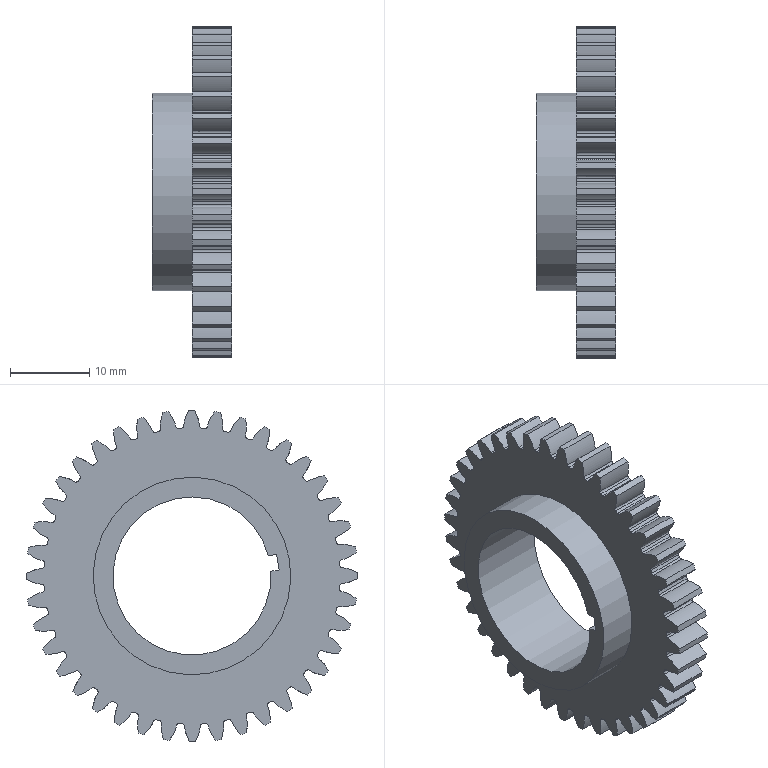Component | NX | SHE_JI-5 | 1 solid | 248 faces | volume 5526 mm3 | other 160 | cylinder 82 | plane 6 | commonest cylinder face diameters 37.5 x40 42 x40 25 x1 20 x1